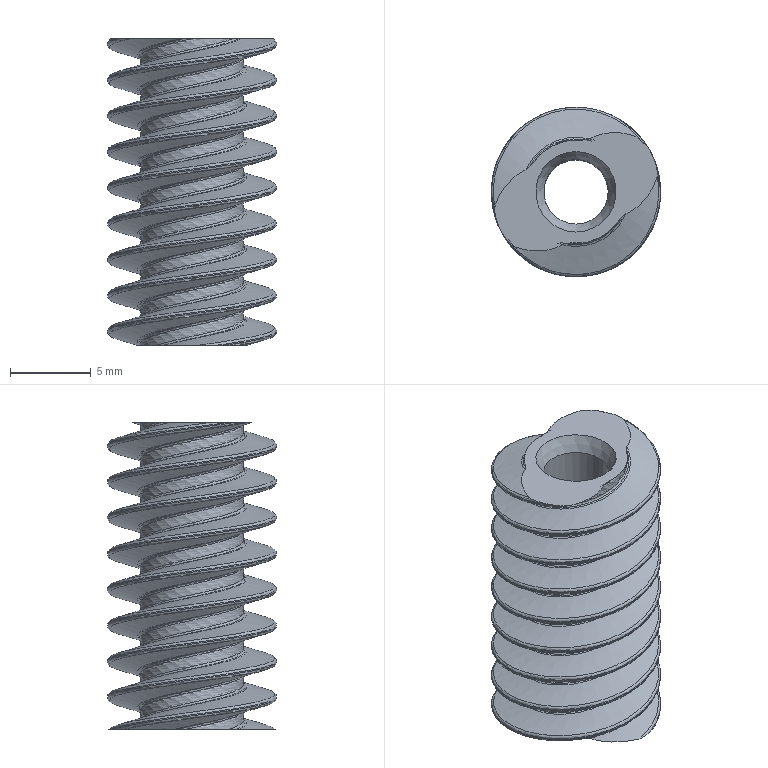CAM job | NX | mm | simultaneous | 1 set-up | 10 operations | part box 10.49 x 10.49 x 19
set-up 1
1. Variable-axis Surface Contouring | Mill Mill5 D1R0.2 | PROFILE_3D_COPY_1 | path 3790.509 mm | 1.665 min
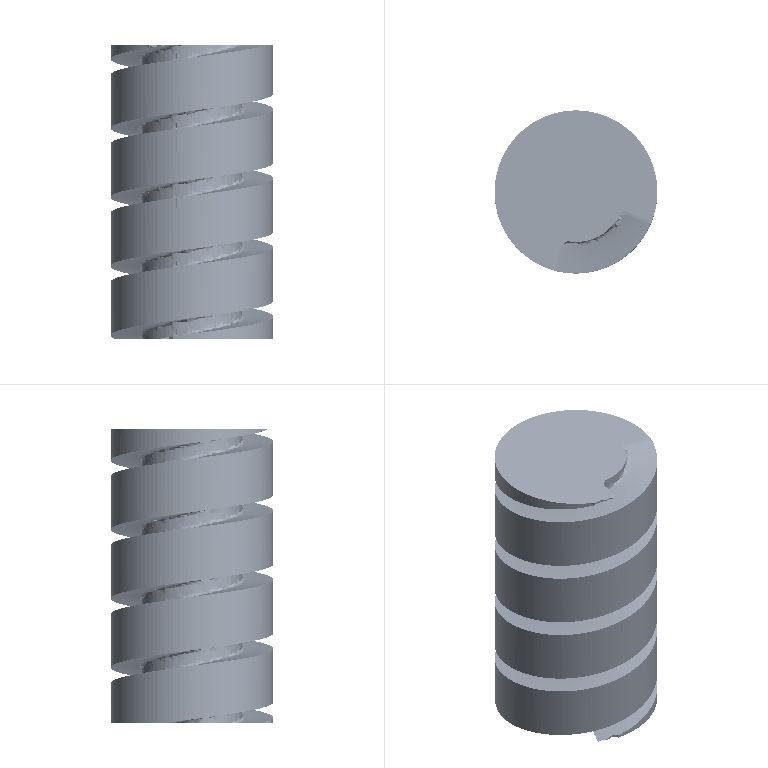2. Variable-axis Surface Contouring | Mill Mill5 D1R0.2 | PROFILE_3D_COPY_1_INSTANCE | path 3790.509 mm | 1.665 min
3. Variable-axis Surface Contouring | Mill Mill5 R0.5 | VARIABLE_STREAMLINE_COPY_COPY | path 8149.534 mm | 4.522 min
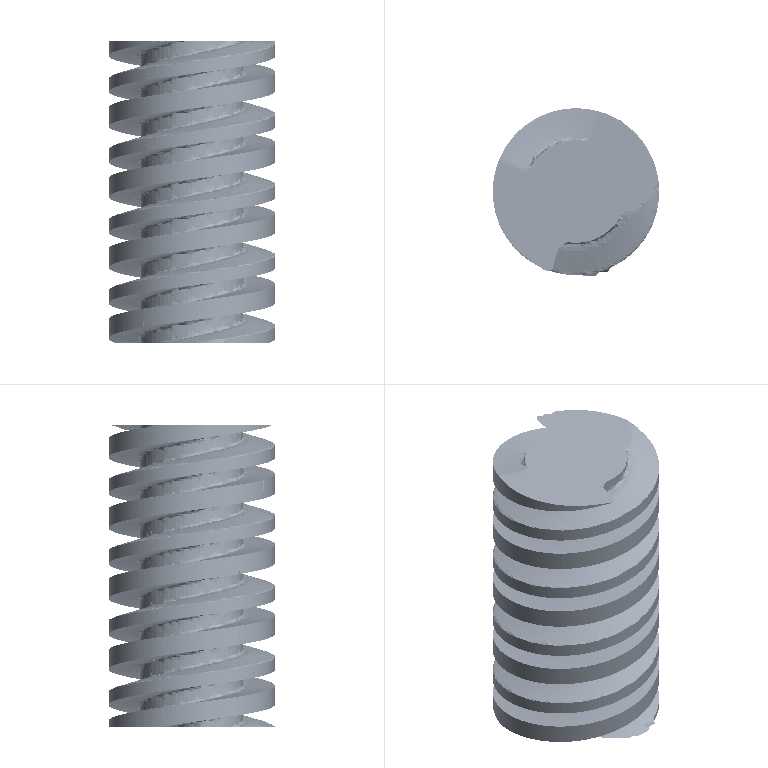4. Variable-axis Surface Contouring | Mill Mill5 R0.5 | VARIABLE_STREAMLINE_COPY_COPY_COPY | path 7361.93 mm | 4.063 min
5. Variable-axis Surface Contouring | Mill Mill5 R0.5 | VARIABLE_STREAMLINE_COPY_COPY_INSTANCE | path 8149.534 mm | 4.522 min
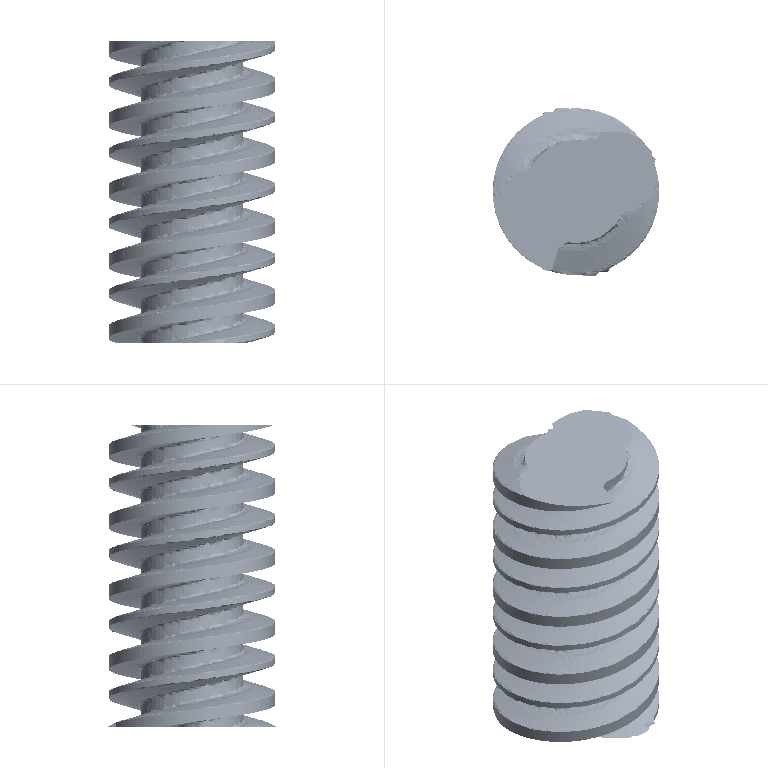6. Variable-axis Surface Contouring | Mill Mill5 R0.5 | VARIABLE_STREAMLINE_COPY_COPY_COPY_INSTANCE | path 7361.93 mm | 4.063 min
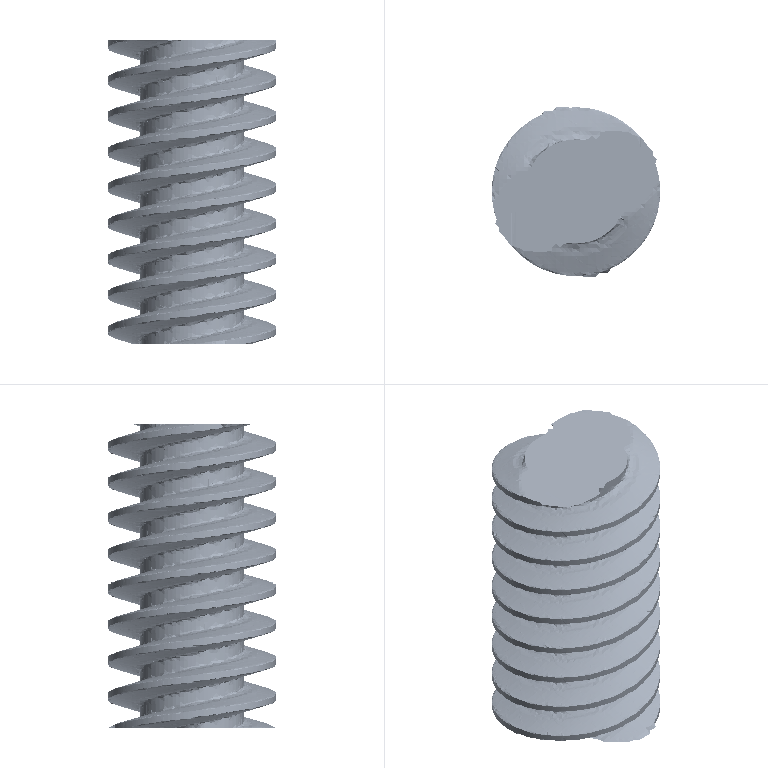7. Variable-axis Surface Contouring | Mill Mill5 R0.5 | VARIABLE_STREAMLINE_COPY_2_COPY | path 12524.903 mm | 6.951 min
8. Variable-axis Surface Contouring | Mill Mill5 R0.5 | VARIABLE_STREAMLINE_COPY_COPY_1_COPY | path 15632.679 mm | 8.677 min
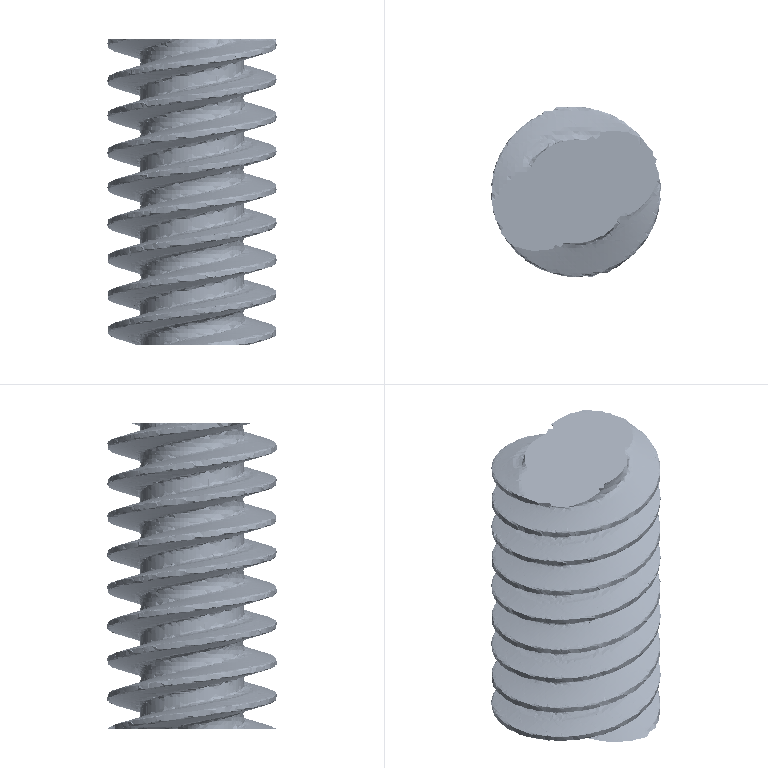9. Variable-axis Surface Contouring | Mill Mill5 R0.5 | VARIABLE_STREAMLINE_COPY_2_COPY_INSTANCE | path 12524.903 mm | 6.951 min
10. Variable-axis Surface Contouring | Mill Mill5 R0.5 | VARIABLE_STREAMLINE_COPY_COPY_1_COPY_INSTANCE | path 15632.679 mm | 8.677 min